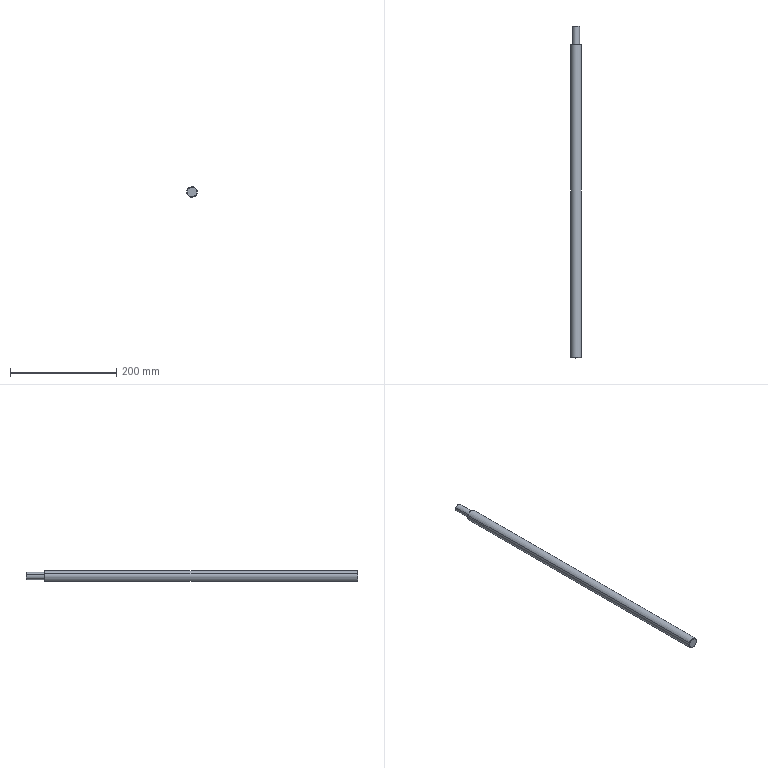Component | SolidWorks | YC1-250-04BalancerAssembly#16673-1_YC1-250-04-10Double-endedScrew#16673-1 | 1 solid | 9 faces | box 20 x 625 x 20 mm | volume 190368 mm3 | cylinder 4 | plane 3 | cone 2 | commonest cylinder face diameters 13.546 x2 20 x2 | material Plain Carbon Steel
STEP:
#1=COLOUR_RGB('',0.7922,0.8196,0.9333);
#2=FILL_AREA_STYLE_COLOUR('',#1);
#3=FILL_AREA_STYLE('',(#2));
#4=SURFACE_STYLE_FILL_AREA(#3);
#5=SURFACE_SIDE_STYLE('',(#4));
#6=SURFACE_STYLE_USAGE(.BOTH.,#5);
#7=PRESENTATION_STYLE_ASSIGNMENT((#6));
#8=CARTESIAN_POINT('',(-13.617,179.724,-4.615));
#9=VERTEX_POINT('',#8);
#10=CARTESIAN_POINT('',(-13.138,179.724,-4.85));
#11=VERTEX_POINT('',#10);
#12=CARTESIAN_POINT('',(-13.378,179.724,-4.733));
#13=DIRECTION('',(0.,1.,-0.));
#14=DIRECTION('',(-0.8982,0.,0.4395));
#15=AXIS2_PLACEMENT_3D('',#12,#13,#14);
#16=CIRCLE('',#15,0.2667);
#17=EDGE_CURVE('',#9,#11,#16,.T.);
#18=ORIENTED_EDGE('',*,*,#17,.T.);
#19=CARTESIAN_POINT('',(-13.138,181.102,-4.85));
#20=VERTEX_POINT('',#19);
#21=CARTESIAN_POINT('',(-13.138,181.791,-4.85));
#22=DIRECTION('',(0.,1.,-0.));
#23=VECTOR('',#22,39.37);
#24=LINE('',#21,#23);
#25=EDGE_CURVE('',#11,#20,#24,.T.);
#26=ORIENTED_EDGE('',*,*,#25,.T.);
#27=CARTESIAN_POINT('',(-13.617,181.102,-4.615));
#28=VERTEX_POINT('',#27);
#29=CARTESIAN_POINT('',(-13.378,181.102,-4.733));
#30=DIRECTION('',(0.,1.,-0.));
#31=DIRECTION('',(0.8982,0.,-0.4395));
#32=AXIS2_PLACEMENT_3D('',#29,#30,#31);
#33=CIRCLE('',#32,0.2667);
#34=EDGE_CURVE('',#28,#20,#33,.T.);
#35=ORIENTED_EDGE('',*,*,#34,.F.);
#36=CARTESIAN_POINT('',(-13.617,181.791,-4.615));
#37=DIRECTION('',(0.,1.,-0.));
#38=VECTOR('',#37,39.37);
#39=LINE('',#36,#38);
#40=EDGE_CURVE('',#9,#28,#39,.T.);
#41=ORIENTED_EDGE('',*,*,#40,.F.);
#42=EDGE_LOOP('',(#18,#26,#35,#41));
#43=FACE_OUTER_BOUND('',#42,.T.);
#44=CARTESIAN_POINT('',(-13.378,181.791,-4.733));
#45=DIRECTION('',(0.,1.,-0.));
#46=DIRECTION('',(-0.8982,0.,0.4395));
#47=AXIS2_PLACEMENT_3D('',#44,#45,#46);
#48=CYLINDRICAL_SURFACE('',#47,0.2667);
#49=ADVANCED_FACE('',(#43),#48,.T.);
#50=CARTESIAN_POINT('',(-13.731,156.535,-4.56));
#51=VERTEX_POINT('',#50);
#52=CARTESIAN_POINT('',(-13.024,156.535,-4.906));
#53=VERTEX_POINT('',#52);
#54=CARTESIAN_POINT('',(-13.378,156.535,-4.733));
#55=DIRECTION('',(0.,1.,-0.));
#56=DIRECTION('',(-0.8982,0.,0.4395));
#57=AXIS2_PLACEMENT_3D('',#54,#55,#56);
#58=CIRCLE('',#57,0.3937);
#59=EDGE_CURVE('',#51,#53,#58,.T.);
#60=ORIENTED_EDGE('',*,*,#59,.T.);
#61=CARTESIAN_POINT('',(-13.024,179.724,-4.906));
#62=VERTEX_POINT('',#61);
#63=CARTESIAN_POINT('',(-13.024,156.496,-4.906));
#64=DIRECTION('',(0.,1.,-0.));
#65=VECTOR('',#64,39.37);
#66=LINE('',#63,#65);
#67=EDGE_CURVE('',#53,#62,#66,.T.);
#68=ORIENTED_EDGE('',*,*,#67,.T.);
#69=CARTESIAN_POINT('',(-13.731,179.724,-4.56));
#70=VERTEX_POINT('',#69);
#71=CARTESIAN_POINT('',(-13.378,179.724,-4.733));
#72=DIRECTION('',(0.,1.,-0.));
#73=DIRECTION('',(0.8982,0.,-0.4395));
#74=AXIS2_PLACEMENT_3D('',#71,#72,#73);
#75=CIRCLE('',#74,0.3937);
#76=EDGE_CURVE('',#70,#62,#75,.T.);
#77=ORIENTED_EDGE('',*,*,#76,.F.);
#78=CARTESIAN_POINT('',(-13.731,156.496,-4.56));
#79=DIRECTION('',(0.,1.,-0.));
#80=VECTOR('',#79,39.37);
#81=LINE('',#78,#80);
#82=EDGE_CURVE('',#51,#70,#81,.T.);
#83=ORIENTED_EDGE('',*,*,#82,.F.);
#84=EDGE_LOOP('',(#60,#68,#77,#83));
#85=FACE_OUTER_BOUND('',#84,.T.);
#86=CARTESIAN_POINT('',(-13.378,156.496,-4.733));
#87=DIRECTION('',(0.,1.,-0.));
#88=DIRECTION('',(-0.8982,0.,0.4395));
#89=AXIS2_PLACEMENT_3D('',#86,#87,#88);
#90=CYLINDRICAL_SURFACE('',#89,0.3937);
#91=ADVANCED_FACE('',(#85),#90,.T.);
#92=CARTESIAN_POINT('',(-13.696,156.496,-4.577));
#93=VERTEX_POINT('',#92);
#94=CARTESIAN_POINT('',(-13.059,156.496,-4.888));
#95=VERTEX_POINT('',#94);
#96=CARTESIAN_POINT('',(-13.378,156.496,-4.733));
#97=DIRECTION('',(0.,1.,-0.));
#98=DIRECTION('',(-0.8982,0.,0.4395));
#99=AXIS2_PLACEMENT_3D('',#96,#97,#98);
#100=CIRCLE('',#99,0.3543);
#101=EDGE_CURVE('',#93,#95,#100,.T.);
#102=ORIENTED_EDGE('',*,*,#101,.T.);
#103=CARTESIAN_POINT('',(-13.024,156.535,-4.906));
#104=DIRECTION('',(0.6352,0.7071,-0.3108));
#105=VECTOR('',#104,39.37);
#106=LINE('',#103,#105);
#107=EDGE_CURVE('',#95,#53,#106,.T.);
#108=ORIENTED_EDGE('',*,*,#107,.T.);
#109=ORIENTED_EDGE('',*,*,#59,.F.);
#110=CARTESIAN_POINT('',(-13.731,156.535,-4.56));
#111=DIRECTION('',(-0.6352,0.7071,0.3108));
#112=VECTOR('',#111,39.37);
#113=LINE('',#110,#112);
#114=EDGE_CURVE('',#93,#51,#113,.T.);
#115=ORIENTED_EDGE('',*,*,#114,.F.);
#116=EDGE_LOOP('',(#102,#108,#109,#115));
#117=FACE_OUTER_BOUND('',#116,.T.);
#118=CARTESIAN_POINT('',(-13.378,156.535,-4.733));
#119=DIRECTION('',(0.,1.,-0.));
#120=DIRECTION('',(-0.8982,0.,0.4395));
#121=AXIS2_PLACEMENT_3D('',#118,#119,#120);
#122=CONICAL_SURFACE('',#121,0.3937,0.7854);
#123=ADVANCED_FACE('',(#117),#122,.T.);
#124=ORIENTED_EDGE('',*,*,#67,.F.);
#125=CARTESIAN_POINT('',(-13.378,156.535,-4.733));
#126=DIRECTION('',(0.,1.,-0.));
#127=DIRECTION('',(-0.8982,0.,0.4395));
#128=AXIS2_PLACEMENT_3D('',#125,#126,#127);
#129=CIRCLE('',#128,0.3937);
#130=EDGE_CURVE('',#53,#51,#129,.T.);
#131=ORIENTED_EDGE('',*,*,#130,.T.);
#132=ORIENTED_EDGE('',*,*,#82,.T.);
#133=CARTESIAN_POINT('',(-13.378,179.724,-4.733));
#134=DIRECTION('',(0.,1.,-0.));
#135=DIRECTION('',(0.8982,0.,-0.4395));
#136=AXIS2_PLACEMENT_3D('',#133,#134,#135);
#137=CIRCLE('',#136,0.3937);
#138=EDGE_CURVE('',#62,#70,#137,.T.);
#139=ORIENTED_EDGE('',*,*,#138,.F.);
#140=EDGE_LOOP('',(#124,#131,#132,#139));
#141=FACE_OUTER_BOUND('',#140,.T.);
#142=CARTESIAN_POINT('',(-13.378,156.496,-4.733));
#143=DIRECTION('',(0.,1.,-0.));
#144=DIRECTION('',(-0.8982,0.,0.4395));
#145=AXIS2_PLACEMENT_3D('',#142,#143,#144);
#146=CYLINDRICAL_SURFACE('',#145,0.3937);
#147=ADVANCED_FACE('',(#141),#146,.T.);
#148=ORIENTED_EDGE('',*,*,#107,.F.);
#149=CARTESIAN_POINT('',(-13.378,156.496,-4.733));
#150=DIRECTION('',(0.,1.,-0.));
#151=DIRECTION('',(-0.8982,0.,0.4395));
#152=AXIS2_PLACEMENT_3D('',#149,#150,#151);
#153=CIRCLE('',#152,0.3543);
#154=EDGE_CURVE('',#95,#93,#153,.T.);
#155=ORIENTED_EDGE('',*,*,#154,.T.);
#156=ORIENTED_EDGE('',*,*,#114,.T.);
#157=ORIENTED_EDGE('',*,*,#130,.F.);
#158=EDGE_LOOP('',(#148,#155,#156,#157));
#159=FACE_OUTER_BOUND('',#158,.T.);
#160=CARTESIAN_POINT('',(-13.378,156.535,-4.733));
#161=DIRECTION('',(0.,1.,-0.));
#162=DIRECTION('',(-0.8982,0.,0.4395));
#163=AXIS2_PLACEMENT_3D('',#160,#161,#162);
#164=CONICAL_SURFACE('',#163,0.3937,0.7854);
#165=ADVANCED_FACE('',(#159),#164,.T.);
#166=ORIENTED_EDGE('',*,*,#101,.F.);
#167=ORIENTED_EDGE('',*,*,#154,.F.);
#168=EDGE_LOOP('',(#166,#167));
#169=FACE_OUTER_BOUND('',#168,.T.);
#170=CARTESIAN_POINT('',(-13.378,156.496,-4.733));
#171=DIRECTION('',(-0.,-1.,0.));
#172=DIRECTION('',(0.8982,-0.,-0.4395));
#173=AXIS2_PLACEMENT_3D('',#170,#171,#172);
#174=PLANE('',#173);
#175=ADVANCED_FACE('',(#169),#174,.T.);
#176=ORIENTED_EDGE('',*,*,#25,.F.);
#177=CARTESIAN_POINT('',(-13.378,179.724,-4.733));
#178=DIRECTION('',(0.,1.,-0.));
#179=DIRECTION('',(-0.8982,0.,0.4395));
#180=AXIS2_PLACEMENT_3D('',#177,#178,#179);
#181=CIRCLE('',#180,0.2667);
#182=EDGE_CURVE('',#11,#9,#181,.T.);
#183=ORIENTED_EDGE('',*,*,#182,.T.);
#184=ORIENTED_EDGE('',*,*,#40,.T.);
#185=CARTESIAN_POINT('',(-13.378,181.102,-4.733));
#186=DIRECTION('',(0.,1.,-0.));
#187=DIRECTION('',(0.8982,0.,-0.4395));
#188=AXIS2_PLACEMENT_3D('',#185,#186,#187);
#189=CIRCLE('',#188,0.2667);
#190=EDGE_CURVE('',#20,#28,#189,.T.);
#191=ORIENTED_EDGE('',*,*,#190,.F.);
#192=EDGE_LOOP('',(#176,#183,#184,#191));
#193=FACE_OUTER_BOUND('',#192,.T.);
#194=CARTESIAN_POINT('',(-13.378,181.791,-4.733));
#195=DIRECTION('',(0.,1.,-0.));
#196=DIRECTION('',(-0.8982,0.,0.4395));
#197=AXIS2_PLACEMENT_3D('',#194,#195,#196);
#198=CYLINDRICAL_SURFACE('',#197,0.2667);
#199=ADVANCED_FACE('',(#193),#198,.T.);
#200=ORIENTED_EDGE('',*,*,#76,.T.);
#201=ORIENTED_EDGE('',*,*,#138,.T.);
#202=EDGE_LOOP('',(#200,#201));
#203=FACE_OUTER_BOUND('',#202,.T.);
#204=ORIENTED_EDGE('',*,*,#17,.F.);
#205=ORIENTED_EDGE('',*,*,#182,.F.);
#206=EDGE_LOOP('',(#204,#205));
#207=FACE_BOUND('',#206,.T.);
#208=CARTESIAN_POINT('',(-13.187,179.724,-4.344));
#209=DIRECTION('',(-0.,-1.,0.));
#210=DIRECTION('',(0.8982,-0.,-0.4395));
#211=AXIS2_PLACEMENT_3D('',#208,#209,#210);
#212=PLANE('',#211);
#213=ADVANCED_FACE('',(#203,#207),#212,.F.);
#214=ORIENTED_EDGE('',*,*,#34,.T.);
#215=ORIENTED_EDGE('',*,*,#190,.T.);
#216=EDGE_LOOP('',(#214,#215));
#217=FACE_OUTER_BOUND('',#216,.T.);
#218=CARTESIAN_POINT('',(-13.378,181.102,-4.733));
#219=DIRECTION('',(-0.,-1.,0.));
#220=DIRECTION('',(0.8982,-0.,-0.4395));
#221=AXIS2_PLACEMENT_3D('',#218,#219,#220);
#222=PLANE('',#221);
#223=ADVANCED_FACE('',(#217),#222,.F.);
#224=CLOSED_SHELL('',(#49,#91,#123,#147,#165,#175,#199,#213,#223));
#225=MANIFOLD_SOLID_BREP('',#224);
#226=STYLED_ITEM('',(#7),#225);
#227=(LENGTH_UNIT()NAMED_UNIT(*)SI_UNIT($,.METRE.));
#228=LENGTH_MEASURE_WITH_UNIT(LENGTH_MEASURE(0.0254),#227);
#229=DIMENSIONAL_EXPONENTS(1.,0.,0.,0.,0.,0.,0.);
#230=(CONVERSION_BASED_UNIT('',#228)LENGTH_UNIT()NAMED_UNIT(#229));
#231=UNCERTAINTY_MEASURE_WITH_UNIT(LENGTH_MEASURE(0.00001),#230,'','');
#232=(NAMED_UNIT(*)PLANE_ANGLE_UNIT()SI_UNIT($,.RADIAN.));
#233=(NAMED_UNIT(*)SI_UNIT($,.STERADIAN.)SOLID_ANGLE_UNIT());
#234=(GEOMETRIC_REPRESENTATION_CONTEXT(3)GLOBAL_UNCERTAINTY_ASSIGNED_CONTEXT((#231))GLOBAL_UNIT_ASSIGNED_CONTEXT((#230,#232,#233))REPRESENTATION_CONTEXT('',''));
#235=MECHANICAL_DESIGN_GEOMETRIC_PRESENTATION_REPRESENTATION('',(#226),#234);
#236=PRESENTATION_LAYER_ASSIGNMENT('','',(#226));
#237=CARTESIAN_POINT('',(0.,0.,0.));
#238=DIRECTION('',(0.,0.,1.));
#239=DIRECTION('',(1.,0.,0.));
#240=AXIS2_PLACEMENT_3D('',#237,#238,#239);
#241=(LENGTH_UNIT()NAMED_UNIT(*)SI_UNIT($,.METRE.));
#242=LENGTH_MEASURE_WITH_UNIT(LENGTH_MEASURE(0.0254),#241);
#243=DIMENSIONAL_EXPONENTS(1.,0.,0.,0.,0.,0.,0.);
#244=(CONVERSION_BASED_UNIT('',#242)LENGTH_UNIT()NAMED_UNIT(#243));
#245=UNCERTAINTY_MEASURE_WITH_UNIT(LENGTH_MEASURE(0.00001),#244,'','');
#246=(NAMED_UNIT(*)PLANE_ANGLE_UNIT()SI_UNIT($,.RADIAN.));
#247=(NAMED_UNIT(*)SI_UNIT($,.STERADIAN.)SOLID_ANGLE_UNIT());
#248=(GEOMETRIC_REPRESENTATION_CONTEXT(3)GLOBAL_UNCERTAINTY_ASSIGNED_CONTEXT((#245))GLOBAL_UNIT_ASSIGNED_CONTEXT((#244,#246,#247))REPRESENTATION_CONTEXT('',''));
#249=ADVANCED_BREP_SHAPE_REPRESENTATION('',(#225,#240),#248);